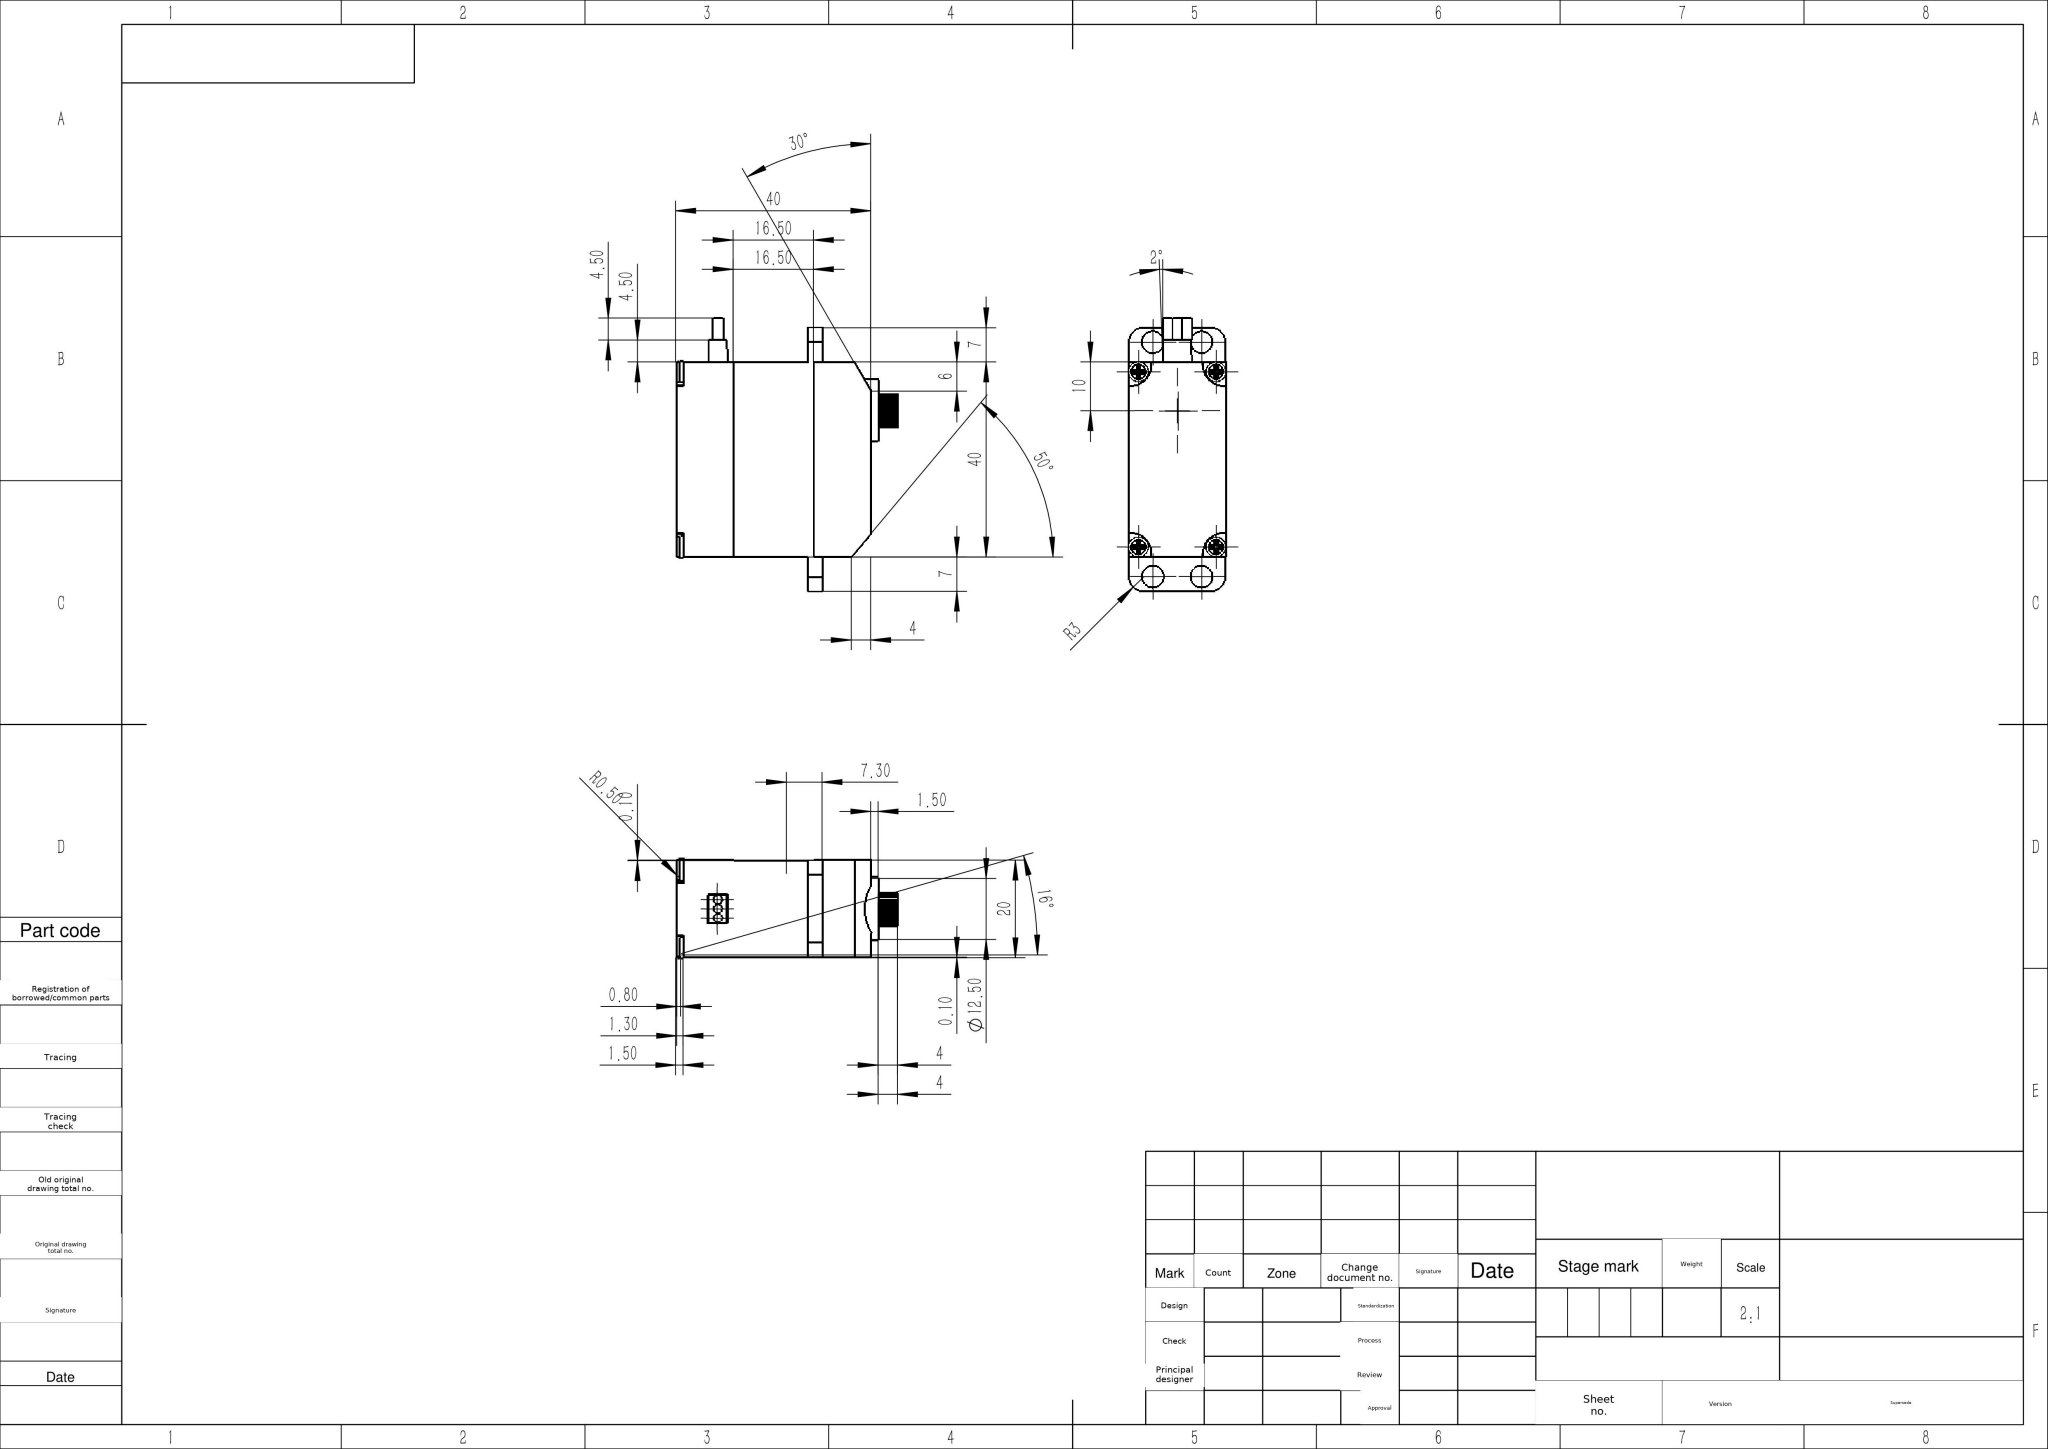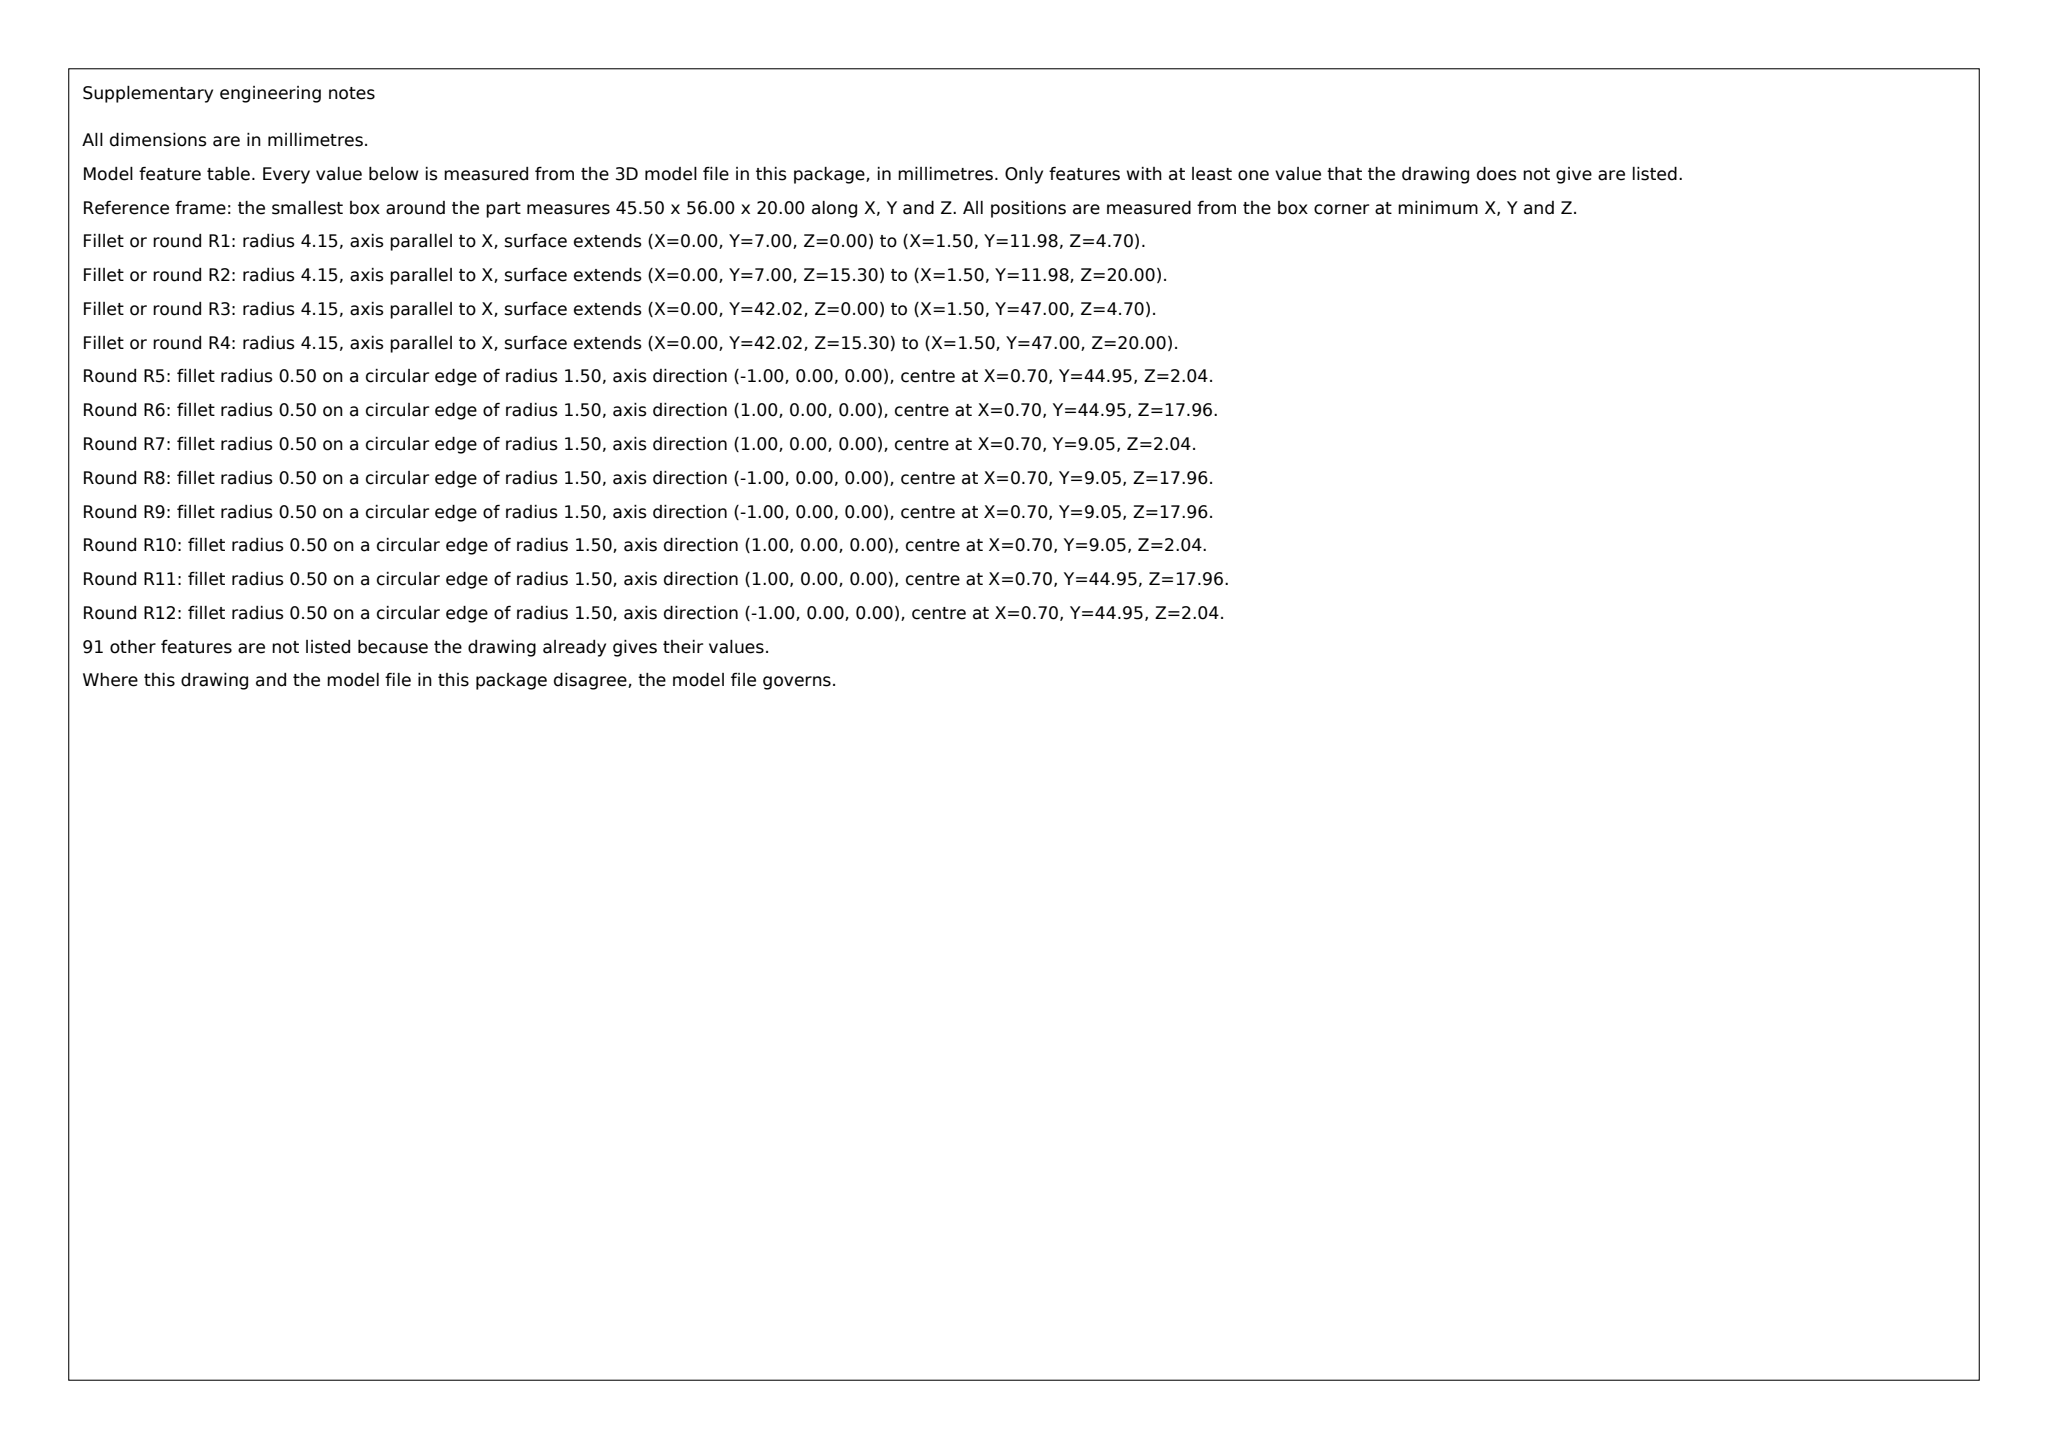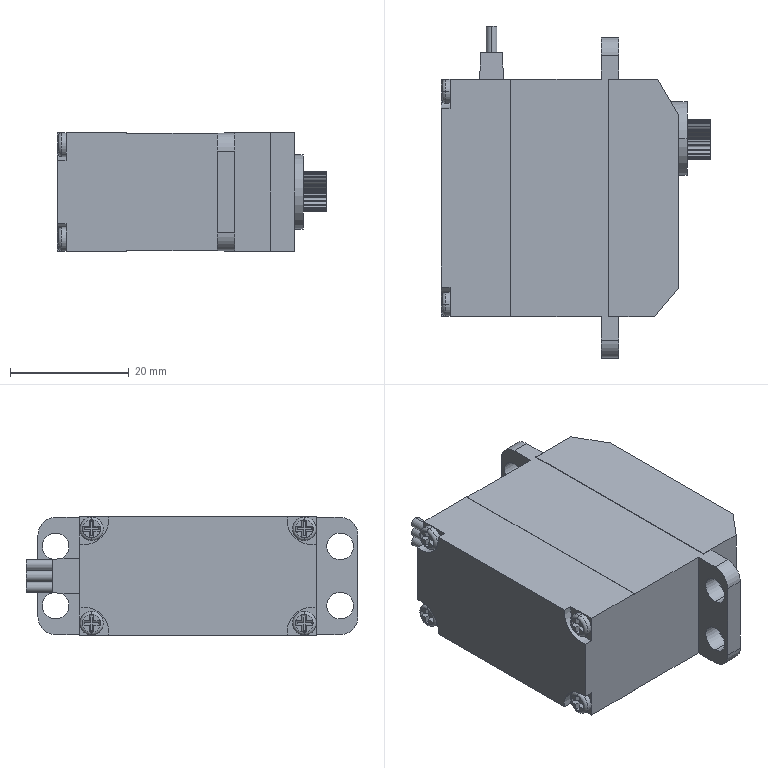Part | SolidWorks | mm | 1 solid | 263 faces | box 45.5 x 56 x 20 mm | volume 32442 mm3 | cylinder 140 | plane 115 | torus 8 | commonest cylinder face diameters 2.5 x54 6.75 x25 5.623 x25 4 x8 4.5 x8 1.8 x6 8.305 x6 6 x4